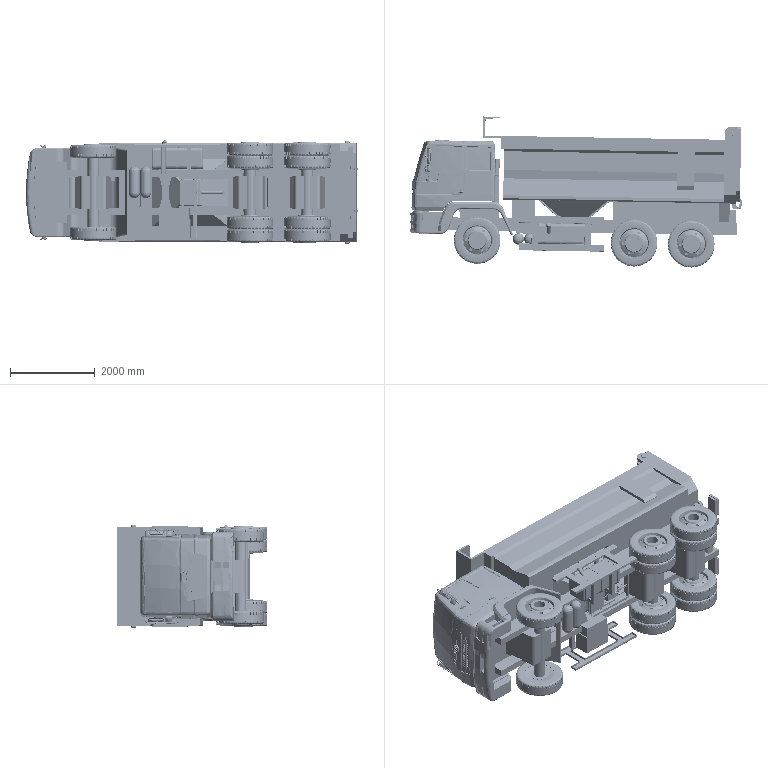Assembly | SolidWorks | mm | 48 component files | 103 solids | 13709 faces | box 7832.96 x 3559.1 x 2433.72 mm | volume 12578933487 mm3 | plane 6009 | cylinder 5038 | sphere 1012 | spline 890 | torus 487 | cone 273 | commonest cylinder face diameters 4 x2056 1069.998 x810 20 x580 50 x184 1 x95 10 x66 6 x66 31.5 x64
Bill of materials:
BoxDoor | 1 |  | Thin flat rectangular plate with two chamfered corners on one long edge and small chamfers on the opposite corners; two small offset tabs, each with one round through-hole, stick out from one edge.
BoxDoorCard | 2 |  | Flat lever or link plate with an irregular outline, extruded to a constant thickness. It has two round through-holes in rounded lobes at one end and a long arm ending in a slanted, pointed tip.
CargoBox | 1 |  | Open, sheet-metal-like rectangular box or frame with a large rectangular window in one side wall. A bent flange or hook sticks out at the top of one end, and the other open end has small pin and hinge-knuckle features with a thin vertical rod.
Front-Lower | 1 |  | Long, slender, ladder-like frame of thin rails and crossmembers. One end has a raised, rounded, hood-like section, and several vertical cylindrical posts and block features hang down along its length.
Front-Upper | 1 |  | Hollow-looking boxy shell with rounded edges. It has a stepped profile, a curved notch or recess on one lower side, embossed rectangular window-like outlines on the side faces, a small handle-like feature, and a thin bent wire loop on top.
RearviewMirror | 2 |  | Elongated rounded-rectangle domed body with a thin flat flange or base plate, and a short cylindrical stem with a rounded end sticking out at an angle from the domed side.
RearviewMirror2 | 2 |  | Near-square rounded body, domed on one side with a thin flat flange on the other, and an angled cylindrical stem with a rounded end sticking out from the dome.
Tire-1 | 10 |  | Wheel-and-tire shaped solid of revolution: a wide toroidal tire-like outer ring with rounded shoulders and short transverse tread lugs/grooves around both shoulder edges, enclosing a recessed dish-shaped rim face with a raised central hub boss, a large central through-bore, and six small circular recesses on a bolt-circle pattern.
FuelTank | 1 |  | Elongated box-shaped vessel with rounded edges and rounded-square ends, raised circumferential bands near both ends and in the middle, and a cylindrical neck or tube sticking out at an angle from the top surface.
'-_-_.STEP_2 | 1 |  | Thin rectangular panel or slab with a narrow stepped strip along one long edge, short cylindrical pins sticking out from the top and bottom edges, and two small apertured tabs on one side face.
'-_-_.STEP | 1 |  | Thin-walled pyramidal or truncated hopper funnel with a rectangular top opening tapering to a smaller rectangular bottom outlet. A rectangular outlet frame and parallel rail or channel members sit at the bottom outlet.
'-_-_-4.STEP | 4 |  | Flanged cylindrical bushing: a short cylinder with a concentric through-bore and a larger, thin flange at one end.
F-M16150U.STEP | 1 |  | Rod-end-like part: a rounded eye housing with a spherical-looking inner ball element and bore, a cylindrical shank, a hexagonal or flatted socket end with an internal bore, and a small nipple-shaped feature sticking out from the shank.
F-SC50CA.STEP | 1 |  | Square mounting-plate bracket with a single projecting clevis-style lug. The plate has rounded corners and four counterbored corner holes. A tapered (triangular in side profile) web rises from the plate centre and ends in a cylindrical boss with a through-bore. The boss ends are chamfered.
GB_T276-94_6003-2Z.STEP | 8 |  | Ring-shaped rolling-element bearing form: concentric outer and inner rings separated by an annular gap, with a ring of spherical elements visible in the gap. It has a plain cylindrical bore and outer surface, and flat faces with small edge chamfers.
GB893_2-86_B_35.STEP | 4 |  | Flat, thin, open split ring with a constant-thickness band. The two free ends carry inward-projecting lugs, each with a small round hole. The lugs sit on the inside of the ring, which matches the general form of an internal-type retaining ring.
GB894_1-86_A_17.STEP | 4 |  | Flat, thin, open split ring with a constant-thickness band. Two lugs, each with a small round hole, project outward at the gap. This matches the general form of an external-type retaining ring.
ZR50_[ZR50-S400-T-R5-M5-C5-P1].STEP | 1 |  | Elongated linear-unit assembly. It has a long rectangular extruded body with longitudinal grooves. A front flange plate has four holes, and a cylindrical rod or shaft with a stepped end protrudes from it. A larger rear housing block sits at the other end, with a box-like unit mounted alongside and parallel to the body. Two flexible cables leave this unit and end in multi-pin connector blocks.
RearBracket | 1 |  | Structural I-section member, apparently with more than one body. One is a short I-section segment. The other is a longer I-section segment with top and bottom flanges, two web or stiffener sections creating open bays between them, and an end plate with tapered haunch transitions at the flange ends.
Subframe | 1 |  | Welded-frame-like weldment made of rectangular and square members. Two long parallel rails are joined by two cross members, giving an H or ladder-shaped planar frame. Two square-section vertical posts rise from the frame. The members appear to be hollow or thin-walled sections.
Mates:
1. concentric | CargoBox-1 face at (936.414, 3015.94, 912.614) dir (0, 0, 1) r 40 | BoxDoor-1 face at (936.414, 3015.94, 1112.614) dir (0, 0, -1) r 40
2. width | BoxDoor-1 face at (839.049, 3167.664, 1047.614) dir (0, 0, 1) | BoxDoor-1 face at (839.049, 3167.664, 977.614) dir (0, 0, -1) | CargoBox-1 face at (699.071, 3170.11, 1052.614) dir (0, 0, -1) | CargoBox-1 face at (699.071, 3170.11, 972.614) dir (0, 0, 1)
3. concentric | CargoBox-1 face at (1130.805, 1262.276, 445.114) dir (0, 0, 1) r 10 | BoxDoorCard-1 face at (1130.805, 1262.276, 520.114) dir (0, 0, -1) r 10
4. width | BoxDoorCard-1 face at (1130.805, 1262.276, 520.114) dir (0, 0, 1) | BoxDoorCard-1 face at (1130.805, 1262.276, 470.114) dir (0, 0, -1) | CargoBox-1 face at (1076.687, 1313.229, 465.114) dir (0, 0, 1) | CargoBox-1 face at (1076.687, 1313.229, 525.114) dir (0, 0, -1)
5. coincident | BoxDoor-1 edge at (1143.424, 1412.078, 862.614) dir (0, 0, -1) | BoxDoorCard-1 face at (1144.905, 1474.638, 470.114) dir (-0.9997, 0.02366, 0)
6. width | FuelTank-1 face at (-3663.859, 823.977, 914.114) dir (-0.9998, 0.01747, 0) | FuelTank-1 face at (-2464.042, 803.012, 914.114) dir (0.9998, -0.01747, 0) | Subframe-1 face at (-2354.69, 1051.139, -62.386) dir (0.9998, -0.01747, 0) | Subframe-1 face at (-3764.475, 1075.773, -62.386) dir (-0.9998, 0.01747, 0)
7. width | FuelTank-1 face at (-3663.859, 823.977, 494.114) dir (0, 0, -1) | FuelTank-1 face at (-3663.859, 823.977, 994.114) dir (0, 0, 1) | Subframe-1 face at (-3607.295, 913.002, 1017.614) dir (0, 0, -1) | Front-1/Front-Lower-1 face at (-6077.139, 1046.174, 470.614) dir (0, 0, 1)
8. coincident | Front-1/Front-Lower-1 face at (-3356.245, 398.538, 1070.614) dir (0.01747, 0.9998, 0) | FuelTank-1 face at (-3671.197, 404.041, 574.114) dir (-0.01747, -0.9998, 0)
9. parallel | Front-1/Front-Upper-1 face at (-6632.324, 2868.151, 1182.614) dir (0.01747, 0.9998, 0) | CargoBox-1 face at (-4865.322, 2967.295, 1819.721) dir (0.01747, 0.9998, 0)
10. distance | Subframe-1 face at (-3499.69, 1061.145, 1067.614) dir (0.01747, 0.9998, 0) | Front-1/Front-Lower-1 face at (-6077.139, 1046.174, 470.614) dir (0.01747, 0.9998, 0)
11. coincident | Subframe-1 edge at (-3419.702, 1059.747, 470.614) dir (-0.9998, 0.01747, 0) | Front-1/Front-Lower-1 face at (-6077.139, 1046.174, 470.614) dir (0, 0, 1)
12. distance | CargoBox-1 face at (-4416.264, 2909.441, 1819.721) dir (-0.01747, -0.9998, 0) | Front-1/Front-Upper-1 face at (-6632.324, 2868.151, 1182.614) dir (0.01747, 0.9998, 0)
13. distance | CargoBox-1 face at (-4439.85, 1559.647, -62.386) dir (-0.9998, 0.01747, 0) | Front-1/Front-Upper-1 face at (-4668.175, -59.611, 1182.614) dir (0.9998, -0.01747, 0)
14. coincident | CargoBox-1 face at (759.356, 1468.797, 912.614) dir (0.01747, 0.9998, 0) | HopperAssembly-1/20211103-210426-70669.STEP-1/-_-_-1.STEP-1/-_-_.STEP-1 edge at (-3663.211, 1546.076, 738.041) dir (0.9998, -0.01747, 0)
15. distance | FuelTank-1 face at (-3663.859, 823.977, 914.114) dir (-0.9998, 0.01747, 0) | Front-1/Front-Lower-1 face at (-3446.406, 390.112, 1070.614) dir (-0.9998, 0.01747, 0)
16. width | HopperAssembly-1/20211103-210426-70669.STEP-1/-_-_-1.STEP-1/-_-_.STEP-1 face at (-2988.232, 880.728, 227.614) dir (0, 0, 1) | HopperAssembly-1/20211103-210426-70669.STEP-1/-_-_-1.STEP-1/-_-_.STEP-1 face at (-2568.297, 873.39, -352.386) dir (0, 0, -1) | CargoBox-1 face at (-4496.252, 2910.838, 1112.614) dir (0, 0, 1) | CargoBox-1 face at (-4496.252, 2910.838, -1237.386) dir (0, 0, -1)
17. width | Front-1/Tire-1-1 face at (-5054.942, 497.231, 1087.614) dir (0, 0, 1) | Front-1/Tire-1-2 face at (-5054.942, 497.231, -1212.386) dir (0, 0, -1) | CargoBox-1 face at (-4496.252, 2910.838, -1237.386) dir (0, 0, -1) | CargoBox-1 face at (-4496.252, 2910.838, 1112.614) dir (0, 0, 1)
18. coincident | Front-1/Front-Lower-1 face at (-6077.139, 1046.174, 470.614) dir (0.01747, 0.9998, 0) | RearBracket-1 face at (-3929.399, 1008.645, 287.614) dir (-0.01747, -0.9998, 0)
19. width | RearBracket-1 face at (1062.563, 1363.484, 367.614) dir (0, 0, 1) | RearBracket-1 face at (1062.563, 1363.484, -492.386) dir (0, 0, -1) | Front-1/Front-Lower-1 face at (-6077.139, 1046.174, -595.386) dir (0, 0, -1) | Front-1/Front-Lower-1 face at (-6077.139, 1046.174, 470.614) dir (0, 0, 1)
20. coincident | Front-1/Front-Lower-1 face at (1054.84, 921.551, 470.614) dir (0.9998, -0.01747, 0) | RearBracket-1 face at (1062.563, 1363.484, -412.386) dir (0.9998, -0.01747, 0)
21. distance | HopperAssembly-1/20211103-210426-70669.STEP-1/-_-_-1.STEP-1/-_-_.STEP-1 face at (-1820.612, 734.306, -892.386) dir (0.9998, -0.01747, 0) | Subframe-1 face at (-2610.001, 1035.597, -1192.386) dir (0.9998, -0.01747, 0)
22. parallel | CargoBox-1 face at (1059.31, 1463.556, -62.386) dir (0.9998, -0.01747, 0) | BoxDoor-1 face at (1158.711, 2286.945, -62.386) dir (0.9998, -0.01747, 0)
23. coincident | Front-Upper-1 plane at (333.86, -2082.115, -8.43) dir (0, 0, 1) | Front-Lower-1 plane at (333.86, -2102.115, -8.43) dir (0, 0, 1)
24. distance | Front-Upper-1 plane at (333.86, -2082.115, -8.43) dir (0, 1, 0) | Front-Lower-1 plane at (333.86, -2102.115, -8.43) dir (0, 1, 0)
25. coincident | Front-Upper-1 plane at (333.86, -2082.115, -8.43) dir (1, 0, 0) | Front-Lower-1 plane at (333.86, -2102.115, -8.43) dir (1, 0, 0)
26. concentric | Front-Upper-1 face at (-600.979, 62.355, 1078.682) dir (0, 1, 0) r 10 | RearviewMirror2-1 face at (-600.979, 210.885, 1078.682) dir (0, -1, 0) r 10
27. concentric | Front-Upper-1 face at (-600.979, 62.355, 1078.682) dir (0, 1, 0) r 10 | RearviewMirror-2 face at (-600.979, 610.885, 1078.682) dir (0, -1, 0) r 10
28. concentric | Front-Upper-1 face at (-600.979, 62.355, -1095.542) dir (0, 1, 0) r 10 | RearviewMirror-3 face at (-600.979, 610.885, -1095.542) dir (0, -1, 0) r 10
29. concentric | Front-Upper-1 face at (-600.979, 62.355, -1095.542) dir (0, 1, 0) r 10 | RearviewMirror2-2 face at (-600.979, 60.885, -1095.542) dir (0, 1, 0) r 10
30. angle | Front-Upper-1 face at (1028.86, -2082.115, 1236.57) dir (1, 0, 0) | RearviewMirror-3 face at (-588.942, 580.885, -1011.19) dir (0.6428, 0, 0.766)
31. angle | Front-Upper-1 face at (1028.86, -2082.115, 1236.57) dir (1, 0, 0) | RearviewMirror2-2 face at (-523.318, 90.885, -1085.345) dir (0.866, 0, 0.5)
32. distance | RearviewMirror-3 face at (-526.426, 615.885, -1076.701) dir (0, 1, 0) | Front-Upper-1 face at (-986.14, 810.885, 1236.57) dir (0, 1, 0)
33. distance | RearviewMirror2-2 face at (-531.978, 215.885, -1090.345) dir (0, 1, 0) | Front-Upper-1 face at (-986.14, 810.885, 1236.57) dir (0, 1, 0)
34. angle | Front-Upper-1 face at (1028.86, -2082.115, 1236.57) dir (1, 0, 0) | RearviewMirror-2 face at (-516.627, 580.885, 1066.645) dir (0.766, 0, -0.6428)
35. angle | Front-Upper-1 face at (1028.86, -2082.115, 1236.57) dir (1, 0, 0) | RearviewMirror2-1 face at (-523.318, 180.885, 1068.485) dir (0.866, 0, -0.5)
36. coincident | RearviewMirror-2 face at (-582.138, 615.885, 1004.129) dir (0, 1, 0) | RearviewMirror-3 face at (-526.426, 615.885, -1076.701) dir (0, 1, 0)
37. coincident | RearviewMirror2-1 face at (-601.978, 215.885, 952.242) dir (0, 1, 0) | RearviewMirror2-2 face at (-531.978, 215.885, -1090.345) dir (0, 1, 0)
38. concentric | Front-Lower-1 face at (632.424, -1532.115, 991.57) dir (0, 0, -1) r 135.665 | Tire-1-2 face at (632.424, -1532.115, -828.43) dir (0, 0, -1) r 550
39. concentric | Front-Lower-1 face at (632.424, -1532.115, 991.57) dir (0, 0, -1) r 135.665 | Tire-1-1 face at (632.424, -1532.115, 811.57) dir (0, 0, 1) r 550
40. distance | Tire-1-1 face at (632.424, -1532.115, 1141.57) dir (0, 0, 1) | Tire-1-2 face at (632.424, -1532.115, -1158.43) dir (0, 0, -1)
41. distance | Front-Upper-1 plane at (333.86, -2082.115, -8.43) dir (0, 0, 1) | Tire-1-2 face at (632.424, -1532.115, -1158.43) dir (0, 0, -1)
42. coincident | Tire-1-3 face at (5682.424, -1532.115, -878.43) dir (0, 0, -1) | Tire-1-4 face at (5682.424, -1532.115, -878.43) dir (0, 0, 1)
43. concentric | Tire-1-3 face at (5682.424, -1532.115, -878.43) dir (0, 0, 1) r 550 | Tire-1-4 face at (5682.424, -1532.115, -878.43) dir (0, 0, -1) r 550
44. concentric | Tire-1-5 face at (5682.424, -1532.115, 861.57) dir (0, 0, -1) r 550 | Tire-1-6 face at (5682.424, -1532.115, 861.57) dir (0, 0, 1) r 550
45. coincident | Tire-1-5 face at (5682.424, -1532.115, 861.57) dir (0, 0, 1) | Tire-1-6 face at (5682.424, -1532.115, 861.57) dir (0, 0, -1)
46. distance | Tire-1-4 face at (5682.424, -1532.115, -1208.43) dir (0, 0, -1) | Tire-1-6 face at (5682.424, -1532.115, 1191.57) dir (0, 0, 1)
47. distance | Front-Upper-1 plane at (333.86, -2082.115, -8.43) dir (0, 0, 1) | Tire-1-6 face at (5682.424, -1532.115, 1191.57) dir (0, 0, 1)
48. coincident | Front-Lower-1 axis at (5682.424, -1532.115, 991.57) dir (0, 0, -1) | Tire-1-6 axis at (5682.424, -1532.115, 854.685) dir (0, 0, -1)
49. coincident | Front-Lower-1 axis at (5682.424, -1532.115, 991.57) dir (0, 0, -1) | Tire-1-3 axis at (5682.424, -1532.115, -933.559) dir (0, 0, -1)